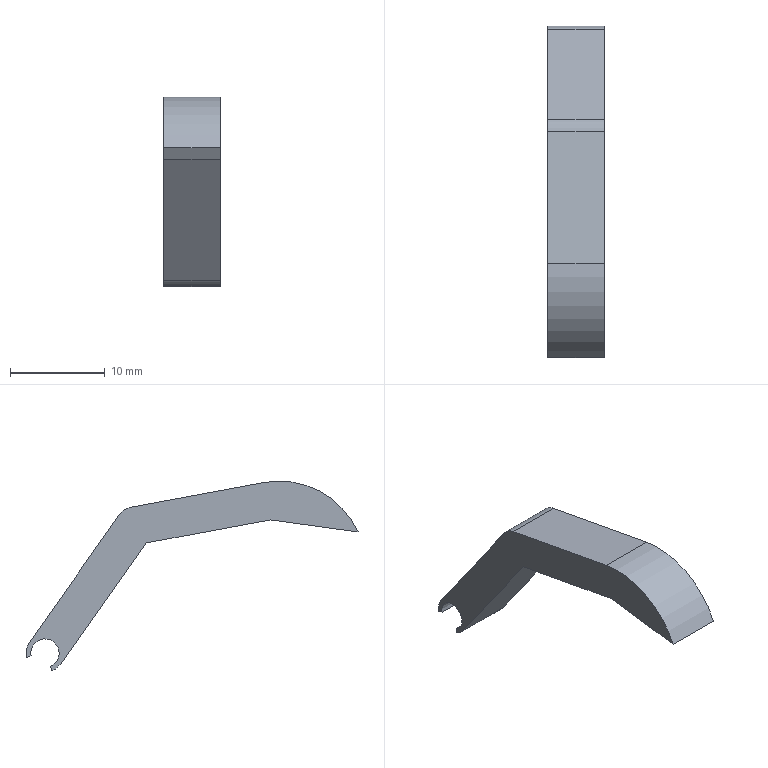Component | SolidWorks | Part14-10 | 1 solid | 17 faces | box 6 x 34.98 x 20 mm | volume 915 mm3 | plane 9 | cylinder 8 | commonest cylinder face diameters 4 x4 3 x3 18.228 x1
STEP:
#1=COLOUR_RGB('',0.7922,0.8196,0.9333);
#2=FILL_AREA_STYLE_COLOUR('',#1);
#3=FILL_AREA_STYLE('',(#2));
#4=SURFACE_STYLE_FILL_AREA(#3);
#5=SURFACE_SIDE_STYLE('',(#4));
#6=SURFACE_STYLE_USAGE(.BOTH.,#5);
#7=PRESENTATION_STYLE_ASSIGNMENT((#6));
#8=CARTESIAN_POINT('',(2.446,-0.3306,0.5502));
#9=VERTEX_POINT('',#8);
#10=CARTESIAN_POINT('',(2.446,-0.3522,0.5709));
#11=VERTEX_POINT('',#10);
#12=CARTESIAN_POINT('',(2.446,-0.2879,0.6163));
#13=DIRECTION('',(-1.,0.,0.));
#14=DIRECTION('',(0.,0.5427,0.84));
#15=AXIS2_PLACEMENT_3D('',#12,#13,#14);
#16=CIRCLE('',#15,0.07874);
#17=EDGE_CURVE('',#9,#11,#16,.T.);
#18=ORIENTED_EDGE('',*,*,#17,.F.);
#19=CARTESIAN_POINT('',(2.682,-0.3306,0.5502));
#20=VERTEX_POINT('',#19);
#21=CARTESIAN_POINT('',(2.446,-0.3306,0.5502));
#22=DIRECTION('',(1.,-0.,-0.));
#23=VECTOR('',#22,39.37);
#24=LINE('',#21,#23);
#25=EDGE_CURVE('',#9,#20,#24,.T.);
#26=ORIENTED_EDGE('',*,*,#25,.T.);
#27=CARTESIAN_POINT('',(2.682,-0.3522,0.5709));
#28=VERTEX_POINT('',#27);
#29=CARTESIAN_POINT('',(2.682,-0.2879,0.6163));
#30=DIRECTION('',(-1.,0.,0.));
#31=DIRECTION('',(0.,0.5427,0.84));
#32=AXIS2_PLACEMENT_3D('',#29,#30,#31);
#33=CIRCLE('',#32,0.07874);
#34=EDGE_CURVE('',#20,#28,#33,.T.);
#35=ORIENTED_EDGE('',*,*,#34,.T.);
#36=CARTESIAN_POINT('',(2.446,-0.3522,0.5709));
#37=DIRECTION('',(1.,-0.,-0.));
#38=VECTOR('',#37,39.37);
#39=LINE('',#36,#38);
#40=EDGE_CURVE('',#11,#28,#39,.T.);
#41=ORIENTED_EDGE('',*,*,#40,.F.);
#42=EDGE_LOOP('',(#18,#26,#35,#41));
#43=FACE_OUTER_BOUND('',#42,.T.);
#44=CARTESIAN_POINT('',(2.446,-0.2879,0.6163));
#45=DIRECTION('',(1.,-0.,-0.));
#46=DIRECTION('',(0.,-0.5427,-0.84));
#47=AXIS2_PLACEMENT_3D('',#44,#45,#46);
#48=CYLINDRICAL_SURFACE('',#47,0.07874);
#49=ADVANCED_FACE('',(#43),#48,.T.);
#50=CARTESIAN_POINT('',(2.446,-0.3199,0.5667));
#51=VERTEX_POINT('',#50);
#52=CARTESIAN_POINT('',(2.446,-0.2558,0.6659));
#53=VERTEX_POINT('',#52);
#54=CARTESIAN_POINT('',(2.446,-0.2879,0.6163));
#55=DIRECTION('',(-1.,0.,0.));
#56=DIRECTION('',(0.,0.5427,0.84));
#57=AXIS2_PLACEMENT_3D('',#54,#55,#56);
#58=CIRCLE('',#57,0.05906);
#59=EDGE_CURVE('',#51,#53,#58,.T.);
#60=ORIENTED_EDGE('',*,*,#59,.T.);
#61=CARTESIAN_POINT('',(2.682,-0.2558,0.6659));
#62=VERTEX_POINT('',#61);
#63=CARTESIAN_POINT('',(2.446,-0.2558,0.6659));
#64=DIRECTION('',(1.,-0.,-0.));
#65=VECTOR('',#64,39.37);
#66=LINE('',#63,#65);
#67=EDGE_CURVE('',#53,#62,#66,.T.);
#68=ORIENTED_EDGE('',*,*,#67,.T.);
#69=CARTESIAN_POINT('',(2.682,-0.3199,0.5667));
#70=VERTEX_POINT('',#69);
#71=CARTESIAN_POINT('',(2.682,-0.2879,0.6163));
#72=DIRECTION('',(-1.,0.,0.));
#73=DIRECTION('',(0.,0.5427,0.84));
#74=AXIS2_PLACEMENT_3D('',#71,#72,#73);
#75=CIRCLE('',#74,0.05906);
#76=EDGE_CURVE('',#70,#62,#75,.T.);
#77=ORIENTED_EDGE('',*,*,#76,.F.);
#78=CARTESIAN_POINT('',(2.446,-0.3199,0.5667));
#79=DIRECTION('',(1.,-0.,-0.));
#80=VECTOR('',#79,39.37);
#81=LINE('',#78,#80);
#82=EDGE_CURVE('',#51,#70,#81,.T.);
#83=ORIENTED_EDGE('',*,*,#82,.F.);
#84=EDGE_LOOP('',(#60,#68,#77,#83));
#85=FACE_OUTER_BOUND('',#84,.T.);
#86=CARTESIAN_POINT('',(2.446,-0.2879,0.6163));
#87=DIRECTION('',(1.,-0.,-0.));
#88=DIRECTION('',(0.,-0.5427,-0.84));
#89=AXIS2_PLACEMENT_3D('',#86,#87,#88);
#90=CYLINDRICAL_SURFACE('',#89,0.05906);
#91=ADVANCED_FACE('',(#85),#90,.F.);
#92=CARTESIAN_POINT('',(2.446,-0.3119,0.5624));
#93=VERTEX_POINT('',#92);
#94=CARTESIAN_POINT('',(2.446,-0.2879,0.6163));
#95=DIRECTION('',(-1.,0.,0.));
#96=DIRECTION('',(0.,0.5427,0.84));
#97=AXIS2_PLACEMENT_3D('',#94,#95,#96);
#98=CIRCLE('',#97,0.05906);
#99=EDGE_CURVE('',#93,#51,#98,.T.);
#100=ORIENTED_EDGE('',*,*,#99,.T.);
#101=ORIENTED_EDGE('',*,*,#82,.T.);
#102=CARTESIAN_POINT('',(2.682,-0.3119,0.5624));
#103=VERTEX_POINT('',#102);
#104=CARTESIAN_POINT('',(2.682,-0.2879,0.6163));
#105=DIRECTION('',(-1.,0.,0.));
#106=DIRECTION('',(0.,0.5427,0.84));
#107=AXIS2_PLACEMENT_3D('',#104,#105,#106);
#108=CIRCLE('',#107,0.05906);
#109=EDGE_CURVE('',#103,#70,#108,.T.);
#110=ORIENTED_EDGE('',*,*,#109,.F.);
#111=CARTESIAN_POINT('',(2.446,-0.3119,0.5624));
#112=DIRECTION('',(1.,-0.,-0.));
#113=VECTOR('',#112,39.37);
#114=LINE('',#111,#113);
#115=EDGE_CURVE('',#93,#103,#114,.T.);
#116=ORIENTED_EDGE('',*,*,#115,.F.);
#117=EDGE_LOOP('',(#100,#101,#110,#116));
#118=FACE_OUTER_BOUND('',#117,.T.);
#119=CARTESIAN_POINT('',(2.446,-0.2879,0.6163));
#120=DIRECTION('',(1.,-0.,-0.));
#121=DIRECTION('',(0.,-0.5427,-0.84));
#122=AXIS2_PLACEMENT_3D('',#119,#120,#121);
#123=CYLINDRICAL_SURFACE('',#122,0.05906);
#124=ADVANCED_FACE('',(#118),#123,.F.);
#125=CARTESIAN_POINT('',(2.682,-0.6463,1.222));
#126=VERTEX_POINT('',#125);
#127=CARTESIAN_POINT('',(2.682,-1.194,1.324));
#128=VERTEX_POINT('',#127);
#129=CARTESIAN_POINT('',(2.682,0.1495,1.074));
#130=DIRECTION('',(-0.,-0.9831,0.183));
#131=VECTOR('',#130,39.37);
#132=LINE('',#129,#131);
#133=EDGE_CURVE('',#126,#128,#132,.T.);
#134=ORIENTED_EDGE('',*,*,#133,.F.);
#135=CARTESIAN_POINT('',(2.446,-0.6463,1.222));
#136=VERTEX_POINT('',#135);
#137=CARTESIAN_POINT('',(2.446,-0.6463,1.222));
#138=DIRECTION('',(1.,-0.,-0.));
#139=VECTOR('',#138,39.37);
#140=LINE('',#137,#139);
#141=EDGE_CURVE('',#136,#126,#140,.T.);
#142=ORIENTED_EDGE('',*,*,#141,.F.);
#143=CARTESIAN_POINT('',(2.446,-1.194,1.324));
#144=VERTEX_POINT('',#143);
#145=CARTESIAN_POINT('',(2.446,0.1495,1.074));
#146=DIRECTION('',(-0.,-0.9831,0.183));
#147=VECTOR('',#146,39.37);
#148=LINE('',#145,#147);
#149=EDGE_CURVE('',#136,#144,#148,.T.);
#150=ORIENTED_EDGE('',*,*,#149,.T.);
#151=CARTESIAN_POINT('',(2.446,-1.194,1.324));
#152=DIRECTION('',(1.,-0.,-0.));
#153=VECTOR('',#152,39.37);
#154=LINE('',#151,#153);
#155=EDGE_CURVE('',#144,#128,#154,.T.);
#156=ORIENTED_EDGE('',*,*,#155,.T.);
#157=EDGE_LOOP('',(#134,#142,#150,#156));
#158=FACE_OUTER_BOUND('',#157,.T.);
#159=CARTESIAN_POINT('',(2.446,0.1495,1.074));
#160=DIRECTION('',(0.,0.183,0.9831));
#161=DIRECTION('',(0.,0.9831,-0.183));
#162=AXIS2_PLACEMENT_3D('',#159,#160,#161);
#163=PLANE('',#162);
#164=ADVANCED_FACE('',(#158),#163,.T.);
#165=CARTESIAN_POINT('',(2.682,-0.5963,1.19));
#166=VERTEX_POINT('',#165);
#167=CARTESIAN_POINT('',(2.682,-0.6607,1.145));
#168=DIRECTION('',(-1.,0.,0.));
#169=DIRECTION('',(0.,0.5427,0.84));
#170=AXIS2_PLACEMENT_3D('',#167,#168,#169);
#171=CIRCLE('',#170,0.07874);
#172=EDGE_CURVE('',#126,#166,#171,.T.);
#173=ORIENTED_EDGE('',*,*,#172,.T.);
#174=CARTESIAN_POINT('',(2.446,-0.5963,1.19));
#175=VERTEX_POINT('',#174);
#176=CARTESIAN_POINT('',(2.446,-0.5963,1.19));
#177=DIRECTION('',(1.,-0.,-0.));
#178=VECTOR('',#177,39.37);
#179=LINE('',#176,#178);
#180=EDGE_CURVE('',#175,#166,#179,.T.);
#181=ORIENTED_EDGE('',*,*,#180,.F.);
#182=CARTESIAN_POINT('',(2.446,-0.6607,1.145));
#183=DIRECTION('',(-1.,0.,0.));
#184=DIRECTION('',(0.,0.5427,0.84));
#185=AXIS2_PLACEMENT_3D('',#182,#183,#184);
#186=CIRCLE('',#185,0.07874);
#187=EDGE_CURVE('',#136,#175,#186,.T.);
#188=ORIENTED_EDGE('',*,*,#187,.F.);
#189=ORIENTED_EDGE('',*,*,#141,.T.);
#190=EDGE_LOOP('',(#173,#181,#188,#189));
#191=FACE_OUTER_BOUND('',#190,.T.);
#192=CARTESIAN_POINT('',(2.446,-0.6607,1.145));
#193=DIRECTION('',(1.,-0.,-0.));
#194=DIRECTION('',(0.,-0.5427,-0.84));
#195=AXIS2_PLACEMENT_3D('',#192,#193,#194);
#196=CYLINDRICAL_SURFACE('',#195,0.07874);
#197=ADVANCED_FACE('',(#191),#196,.T.);
#198=CARTESIAN_POINT('',(2.682,-0.2235,0.6617));
#199=VERTEX_POINT('',#198);
#200=CARTESIAN_POINT('',(2.682,0.241,0.003505));
#201=DIRECTION('',(0.,-0.5766,0.817));
#202=VECTOR('',#201,39.37);
#203=LINE('',#200,#202);
#204=EDGE_CURVE('',#199,#166,#203,.T.);
#205=ORIENTED_EDGE('',*,*,#204,.F.);
#206=CARTESIAN_POINT('',(2.446,-0.2235,0.6617));
#207=VERTEX_POINT('',#206);
#208=CARTESIAN_POINT('',(2.446,-0.2235,0.6617));
#209=DIRECTION('',(1.,-0.,-0.));
#210=VECTOR('',#209,39.37);
#211=LINE('',#208,#210);
#212=EDGE_CURVE('',#207,#199,#211,.T.);
#213=ORIENTED_EDGE('',*,*,#212,.F.);
#214=CARTESIAN_POINT('',(2.446,0.241,0.003505));
#215=DIRECTION('',(0.,-0.5766,0.817));
#216=VECTOR('',#215,39.37);
#217=LINE('',#214,#216);
#218=EDGE_CURVE('',#207,#175,#217,.T.);
#219=ORIENTED_EDGE('',*,*,#218,.T.);
#220=ORIENTED_EDGE('',*,*,#180,.T.);
#221=EDGE_LOOP('',(#205,#213,#219,#220));
#222=FACE_OUTER_BOUND('',#221,.T.);
#223=CARTESIAN_POINT('',(2.446,0.241,0.003505));
#224=DIRECTION('',(0.,0.817,0.5766));
#225=DIRECTION('',(-0.,0.5766,-0.817));
#226=AXIS2_PLACEMENT_3D('',#223,#224,#225);
#227=PLANE('',#226);
#228=ADVANCED_FACE('',(#222),#227,.T.);
#229=CARTESIAN_POINT('',(2.682,-0.2114,0.5977));
#230=VERTEX_POINT('',#229);
#231=CARTESIAN_POINT('',(2.682,-0.2879,0.6163));
#232=DIRECTION('',(-1.,0.,0.));
#233=DIRECTION('',(0.,0.5427,0.84));
#234=AXIS2_PLACEMENT_3D('',#231,#232,#233);
#235=CIRCLE('',#234,0.07874);
#236=EDGE_CURVE('',#199,#230,#235,.T.);
#237=ORIENTED_EDGE('',*,*,#236,.T.);
#238=CARTESIAN_POINT('',(2.446,-0.2114,0.5977));
#239=VERTEX_POINT('',#238);
#240=CARTESIAN_POINT('',(2.446,-0.2114,0.5977));
#241=DIRECTION('',(1.,-0.,-0.));
#242=VECTOR('',#241,39.37);
#243=LINE('',#240,#242);
#244=EDGE_CURVE('',#239,#230,#243,.T.);
#245=ORIENTED_EDGE('',*,*,#244,.F.);
#246=CARTESIAN_POINT('',(2.446,-0.2879,0.6163));
#247=DIRECTION('',(-1.,0.,0.));
#248=DIRECTION('',(0.,0.5427,0.84));
#249=AXIS2_PLACEMENT_3D('',#246,#247,#248);
#250=CIRCLE('',#249,0.07874);
#251=EDGE_CURVE('',#207,#239,#250,.T.);
#252=ORIENTED_EDGE('',*,*,#251,.F.);
#253=ORIENTED_EDGE('',*,*,#212,.T.);
#254=EDGE_LOOP('',(#237,#245,#252,#253));
#255=FACE_OUTER_BOUND('',#254,.T.);
#256=CARTESIAN_POINT('',(2.446,-0.2879,0.6163));
#257=DIRECTION('',(1.,-0.,-0.));
#258=DIRECTION('',(0.,-0.5427,-0.84));
#259=AXIS2_PLACEMENT_3D('',#256,#257,#258);
#260=CYLINDRICAL_SURFACE('',#259,0.07874);
#261=ADVANCED_FACE('',(#255),#260,.T.);
#262=CARTESIAN_POINT('',(2.682,-0.23,0.6047));
#263=VERTEX_POINT('',#262);
#264=CARTESIAN_POINT('',(2.682,0.1655,0.4558));
#265=DIRECTION('',(0.,0.9359,-0.3522));
#266=VECTOR('',#265,39.37);
#267=LINE('',#264,#266);
#268=EDGE_CURVE('',#263,#230,#267,.T.);
#269=ORIENTED_EDGE('',*,*,#268,.F.);
#270=CARTESIAN_POINT('',(2.446,-0.23,0.6047));
#271=VERTEX_POINT('',#270);
#272=CARTESIAN_POINT('',(2.446,-0.23,0.6047));
#273=DIRECTION('',(1.,-0.,-0.));
#274=VECTOR('',#273,39.37);
#275=LINE('',#272,#274);
#276=EDGE_CURVE('',#271,#263,#275,.T.);
#277=ORIENTED_EDGE('',*,*,#276,.F.);
#278=CARTESIAN_POINT('',(2.446,0.1655,0.4558));
#279=DIRECTION('',(0.,0.9359,-0.3522));
#280=VECTOR('',#279,39.37);
#281=LINE('',#278,#280);
#282=EDGE_CURVE('',#271,#239,#281,.T.);
#283=ORIENTED_EDGE('',*,*,#282,.T.);
#284=ORIENTED_EDGE('',*,*,#244,.T.);
#285=EDGE_LOOP('',(#269,#277,#283,#284));
#286=FACE_OUTER_BOUND('',#285,.T.);
#287=CARTESIAN_POINT('',(2.446,0.1655,0.4558));
#288=DIRECTION('',(-0.,-0.3522,-0.9359));
#289=DIRECTION('',(-0.,-0.9359,0.3522));
#290=AXIS2_PLACEMENT_3D('',#287,#288,#289);
#291=PLANE('',#290);
#292=ADVANCED_FACE('',(#286),#291,.T.);
#293=ORIENTED_EDGE('',*,*,#67,.F.);
#294=CARTESIAN_POINT('',(2.446,-0.2879,0.6163));
#295=DIRECTION('',(-1.,0.,0.));
#296=DIRECTION('',(0.,0.5427,0.84));
#297=AXIS2_PLACEMENT_3D('',#294,#295,#296);
#298=CIRCLE('',#297,0.05906);
#299=EDGE_CURVE('',#53,#271,#298,.T.);
#300=ORIENTED_EDGE('',*,*,#299,.T.);
#301=ORIENTED_EDGE('',*,*,#276,.T.);
#302=CARTESIAN_POINT('',(2.682,-0.2879,0.6163));
#303=DIRECTION('',(-1.,0.,0.));
#304=DIRECTION('',(0.,0.5427,0.84));
#305=AXIS2_PLACEMENT_3D('',#302,#303,#304);
#306=CIRCLE('',#305,0.05906);
#307=EDGE_CURVE('',#62,#263,#306,.T.);
#308=ORIENTED_EDGE('',*,*,#307,.F.);
#309=EDGE_LOOP('',(#293,#300,#301,#308));
#310=FACE_OUTER_BOUND('',#309,.T.);
#311=CARTESIAN_POINT('',(2.446,-0.2879,0.6163));
#312=DIRECTION('',(1.,-0.,-0.));
#313=DIRECTION('',(0.,-0.5427,-0.84));
#314=AXIS2_PLACEMENT_3D('',#311,#312,#313);
#315=CYLINDRICAL_SURFACE('',#314,0.05906);
#316=ADVANCED_FACE('',(#310),#315,.F.);
#317=CARTESIAN_POINT('',(2.682,-0.3156,0.5426));
#318=VERTEX_POINT('',#317);
#319=CARTESIAN_POINT('',(2.682,-0.4486,-0.1662));
#320=DIRECTION('',(-0.,-0.1844,-0.9829));
#321=VECTOR('',#320,39.37);
#322=LINE('',#319,#321);
#323=EDGE_CURVE('',#103,#318,#322,.T.);
#324=ORIENTED_EDGE('',*,*,#323,.T.);
#325=CARTESIAN_POINT('',(2.446,-0.3156,0.5426));
#326=VERTEX_POINT('',#325);
#327=CARTESIAN_POINT('',(2.446,-0.3156,0.5426));
#328=DIRECTION('',(1.,-0.,-0.));
#329=VECTOR('',#328,39.37);
#330=LINE('',#327,#329);
#331=EDGE_CURVE('',#326,#318,#330,.T.);
#332=ORIENTED_EDGE('',*,*,#331,.F.);
#333=CARTESIAN_POINT('',(2.446,-0.4486,-0.1662));
#334=DIRECTION('',(-0.,-0.1844,-0.9829));
#335=VECTOR('',#334,39.37);
#336=LINE('',#333,#335);
#337=EDGE_CURVE('',#93,#326,#336,.T.);
#338=ORIENTED_EDGE('',*,*,#337,.F.);
#339=ORIENTED_EDGE('',*,*,#115,.T.);
#340=EDGE_LOOP('',(#324,#332,#338,#339));
#341=FACE_OUTER_BOUND('',#340,.T.);
#342=CARTESIAN_POINT('',(2.446,-0.4486,-0.1662));
#343=DIRECTION('',(-0.,-0.9829,0.1844));
#344=DIRECTION('',(0.,0.1844,0.9829));
#345=AXIS2_PLACEMENT_3D('',#342,#343,#344);
#346=PLANE('',#345);
#347=ADVANCED_FACE('',(#341),#346,.F.);
#348=ORIENTED_EDGE('',*,*,#25,.F.);
#349=CARTESIAN_POINT('',(2.446,-0.2879,0.6163));
#350=DIRECTION('',(-1.,0.,0.));
#351=DIRECTION('',(0.,0.5427,0.84));
#352=AXIS2_PLACEMENT_3D('',#349,#350,#351);
#353=CIRCLE('',#352,0.07874);
#354=EDGE_CURVE('',#326,#9,#353,.T.);
#355=ORIENTED_EDGE('',*,*,#354,.F.);
#356=ORIENTED_EDGE('',*,*,#331,.T.);
#357=CARTESIAN_POINT('',(2.682,-0.2879,0.6163));
#358=DIRECTION('',(-1.,0.,0.));
#359=DIRECTION('',(0.,0.5427,0.84));
#360=AXIS2_PLACEMENT_3D('',#357,#358,#359);
#361=CIRCLE('',#360,0.07874);
#362=EDGE_CURVE('',#318,#20,#361,.T.);
#363=ORIENTED_EDGE('',*,*,#362,.T.);
#364=EDGE_LOOP('',(#348,#355,#356,#363));
#365=FACE_OUTER_BOUND('',#364,.T.);
#366=CARTESIAN_POINT('',(2.446,-0.2879,0.6163));
#367=DIRECTION('',(1.,-0.,-0.));
#368=DIRECTION('',(0.,-0.5427,-0.84));
#369=AXIS2_PLACEMENT_3D('',#366,#367,#368);
#370=CYLINDRICAL_SURFACE('',#369,0.07874);
#371=ADVANCED_FACE('',(#365),#370,.T.);
#372=CARTESIAN_POINT('',(2.682,-0.7066,1.073));
#373=VERTEX_POINT('',#372);
#374=CARTESIAN_POINT('',(2.682,0.1124,-0.0873));
#375=DIRECTION('',(0.,-0.5766,0.817));
#376=VECTOR('',#375,39.37);
#377=LINE('',#374,#376);
#378=EDGE_CURVE('',#28,#373,#377,.T.);
#379=ORIENTED_EDGE('',*,*,#378,.T.);
#380=CARTESIAN_POINT('',(2.446,-0.7066,1.073));
#381=VERTEX_POINT('',#380);
#382=CARTESIAN_POINT('',(2.446,-0.7066,1.073));
#383=DIRECTION('',(1.,-0.,-0.));
#384=VECTOR('',#383,39.37);
#385=LINE('',#382,#384);
#386=EDGE_CURVE('',#381,#373,#385,.T.);
#387=ORIENTED_EDGE('',*,*,#386,.F.);
#388=CARTESIAN_POINT('',(2.446,0.1124,-0.0873));
#389=DIRECTION('',(0.,-0.5766,0.817));
#390=VECTOR('',#389,39.37);
#391=LINE('',#388,#390);
#392=EDGE_CURVE('',#11,#381,#391,.T.);
#393=ORIENTED_EDGE('',*,*,#392,.F.);
#394=ORIENTED_EDGE('',*,*,#40,.T.);
#395=EDGE_LOOP('',(#379,#387,#393,#394));
#396=FACE_OUTER_BOUND('',#395,.T.);
#397=CARTESIAN_POINT('',(2.446,0.1124,-0.0873));
#398=DIRECTION('',(0.,0.817,0.5766));
#399=DIRECTION('',(-0.,0.5766,-0.817));
#400=AXIS2_PLACEMENT_3D('',#397,#398,#399);
#401=PLANE('',#400);
#402=ADVANCED_FACE('',(#396),#401,.F.);
#403=CARTESIAN_POINT('',(2.682,-1.223,1.169));
#404=VERTEX_POINT('',#403);
#405=CARTESIAN_POINT('',(2.682,0.1207,0.9191));
#406=DIRECTION('',(-0.,-0.9831,0.183));
#407=VECTOR('',#406,39.37);
#408=LINE('',#405,#407);
#409=EDGE_CURVE('',#373,#404,#408,.T.);
#410=ORIENTED_EDGE('',*,*,#409,.T.);
#411=CARTESIAN_POINT('',(2.446,-1.223,1.169));
#412=VERTEX_POINT('',#411);
#413=CARTESIAN_POINT('',(2.446,-1.223,1.169));
#414=DIRECTION('',(1.,-0.,-0.));
#415=VECTOR('',#414,39.37);
#416=LINE('',#413,#415);
#417=EDGE_CURVE('',#412,#404,#416,.T.);
#418=ORIENTED_EDGE('',*,*,#417,.F.);
#419=CARTESIAN_POINT('',(2.446,0.1207,0.9191));
#420=DIRECTION('',(-0.,-0.9831,0.183));
#421=VECTOR('',#420,39.37);
#422=LINE('',#419,#421);
#423=EDGE_CURVE('',#381,#412,#422,.T.);
#424=ORIENTED_EDGE('',*,*,#423,.F.);
#425=ORIENTED_EDGE('',*,*,#386,.T.);
#426=EDGE_LOOP('',(#410,#418,#424,#425));
#427=FACE_OUTER_BOUND('',#426,.T.);
#428=CARTESIAN_POINT('',(2.446,0.1207,0.9191));
#429=DIRECTION('',(0.,0.183,0.9831));
#430=DIRECTION('',(0.,0.9831,-0.183));
#431=AXIS2_PLACEMENT_3D('',#428,#429,#430);
#432=PLANE('',#431);
#433=ADVANCED_FACE('',(#427),#432,.F.);
#434=CARTESIAN_POINT('',(2.682,-1.586,1.119));
#435=VERTEX_POINT('',#434);
#436=CARTESIAN_POINT('',(2.682,-0.3035,1.295));
#437=DIRECTION('',(-0.,-0.9907,-0.136));
#438=VECTOR('',#437,39.37);
#439=LINE('',#436,#438);
#440=EDGE_CURVE('',#404,#435,#439,.T.);
#441=ORIENTED_EDGE('',*,*,#440,.T.);
#442=CARTESIAN_POINT('',(2.446,-1.586,1.119));
#443=VERTEX_POINT('',#442);
#444=CARTESIAN_POINT('',(2.446,-1.586,1.119));
#445=DIRECTION('',(1.,-0.,-0.));
#446=VECTOR('',#445,39.37);
#447=LINE('',#444,#446);
#448=EDGE_CURVE('',#443,#435,#447,.T.);
#449=ORIENTED_EDGE('',*,*,#448,.F.);
#450=CARTESIAN_POINT('',(2.446,-0.3035,1.295));
#451=DIRECTION('',(-0.,-0.9907,-0.136));
#452=VECTOR('',#451,39.37);
#453=LINE('',#450,#452);
#454=EDGE_CURVE('',#412,#443,#453,.T.);
#455=ORIENTED_EDGE('',*,*,#454,.F.);
#456=ORIENTED_EDGE('',*,*,#417,.T.);
#457=EDGE_LOOP('',(#441,#449,#455,#456));
#458=FACE_OUTER_BOUND('',#457,.T.);
#459=CARTESIAN_POINT('',(2.446,-0.3035,1.295));
#460=DIRECTION('',(0.,-0.136,0.9907));
#461=DIRECTION('',(0.,0.9907,0.136));
#462=AXIS2_PLACEMENT_3D('',#459,#460,#461);
#463=PLANE('',#462);
#464=ADVANCED_FACE('',(#458),#463,.F.);
#465=CARTESIAN_POINT('',(2.682,-1.26,0.9712));
#466=DIRECTION('',(-1.,0.,0.));
#467=DIRECTION('',(0.,0.5427,0.84));
#468=AXIS2_PLACEMENT_3D('',#465,#466,#467);
#469=CIRCLE('',#468,0.3588);
#470=EDGE_CURVE('',#435,#128,#469,.T.);
#471=ORIENTED_EDGE('',*,*,#470,.T.);
#472=ORIENTED_EDGE('',*,*,#155,.F.);
#473=CARTESIAN_POINT('',(2.446,-1.26,0.9712));
#474=DIRECTION('',(-1.,0.,0.));
#475=DIRECTION('',(0.,0.5427,0.84));
#476=AXIS2_PLACEMENT_3D('',#473,#474,#475);
#477=CIRCLE('',#476,0.3588);
#478=EDGE_CURVE('',#443,#144,#477,.T.);
#479=ORIENTED_EDGE('',*,*,#478,.F.);
#480=ORIENTED_EDGE('',*,*,#448,.T.);
#481=EDGE_LOOP('',(#471,#472,#479,#480));
#482=FACE_OUTER_BOUND('',#481,.T.);
#483=CARTESIAN_POINT('',(2.446,-1.26,0.9712));
#484=DIRECTION('',(1.,-0.,-0.));
#485=DIRECTION('',(0.,-0.5427,-0.84));
#486=AXIS2_PLACEMENT_3D('',#483,#484,#485);
#487=CYLINDRICAL_SURFACE('',#486,0.3588);
#488=ADVANCED_FACE('',(#482),#487,.T.);
#489=ORIENTED_EDGE('',*,*,#149,.F.);
#490=ORIENTED_EDGE('',*,*,#187,.T.);
#491=ORIENTED_EDGE('',*,*,#218,.F.);
#492=ORIENTED_EDGE('',*,*,#251,.T.);
#493=ORIENTED_EDGE('',*,*,#282,.F.);
#494=ORIENTED_EDGE('',*,*,#299,.F.);
#495=ORIENTED_EDGE('',*,*,#59,.F.);
#496=ORIENTED_EDGE('',*,*,#99,.F.);
#497=ORIENTED_EDGE('',*,*,#337,.T.);
#498=ORIENTED_EDGE('',*,*,#354,.T.);
#499=ORIENTED_EDGE('',*,*,#17,.T.);
#500=ORIENTED_EDGE('',*,*,#392,.T.);
#501=ORIENTED_EDGE('',*,*,#423,.T.);
#502=ORIENTED_EDGE('',*,*,#454,.T.);
#503=ORIENTED_EDGE('',*,*,#478,.T.);
#504=EDGE_LOOP('',(#489,#490,#491,#492,#493,#494,#495,#496,#497,#498,#499,#500,#501,#502,#503));
#505=FACE_OUTER_BOUND('',#504,.T.);
#506=CARTESIAN_POINT('',(2.446,-0.09369,-0.2327));
#507=DIRECTION('',(-1.,0.,0.));
#508=DIRECTION('',(0.,0.5427,0.84));
#509=AXIS2_PLACEMENT_3D('',#506,#507,#508);
#510=PLANE('',#509);
#511=ADVANCED_FACE('',(#505),#510,.T.);
#512=ORIENTED_EDGE('',*,*,#133,.T.);
#513=ORIENTED_EDGE('',*,*,#470,.F.);
#514=ORIENTED_EDGE('',*,*,#440,.F.);
#515=ORIENTED_EDGE('',*,*,#409,.F.);
#516=ORIENTED_EDGE('',*,*,#378,.F.);
#517=ORIENTED_EDGE('',*,*,#34,.F.);
#518=ORIENTED_EDGE('',*,*,#362,.F.);
#519=ORIENTED_EDGE('',*,*,#323,.F.);
#520=ORIENTED_EDGE('',*,*,#109,.T.);
#521=ORIENTED_EDGE('',*,*,#76,.T.);
#522=ORIENTED_EDGE('',*,*,#307,.T.);
#523=ORIENTED_EDGE('',*,*,#268,.T.);
#524=ORIENTED_EDGE('',*,*,#236,.F.);
#525=ORIENTED_EDGE('',*,*,#204,.T.);
#526=ORIENTED_EDGE('',*,*,#172,.F.);
#527=EDGE_LOOP('',(#512,#513,#514,#515,#516,#517,#518,#519,#520,#521,#522,#523,#524,#525,#526));
#528=FACE_OUTER_BOUND('',#527,.T.);
#529=CARTESIAN_POINT('',(2.682,-0.09369,-0.2327));
#530=DIRECTION('',(-1.,0.,0.));
#531=DIRECTION('',(0.,0.5427,0.84));
#532=AXIS2_PLACEMENT_3D('',#529,#530,#531);
#533=PLANE('',#532);
#534=ADVANCED_FACE('',(#528),#533,.F.);
#535=CLOSED_SHELL('',(#49,#91,#124,#164,#197,#228,#261,#292,#316,#347,#371,#402,#433,#464,#488,#511,#534));
#536=MANIFOLD_SOLID_BREP('',#535);
#537=STYLED_ITEM('',(#7),#536);
#538=(LENGTH_UNIT()NAMED_UNIT(*)SI_UNIT($,.METRE.));
#539=LENGTH_MEASURE_WITH_UNIT(LENGTH_MEASURE(0.0254),#538);
#540=DIMENSIONAL_EXPONENTS(1.,0.,0.,0.,0.,0.,0.);
#541=(CONVERSION_BASED_UNIT('',#539)LENGTH_UNIT()NAMED_UNIT(#540));
#542=UNCERTAINTY_MEASURE_WITH_UNIT(LENGTH_MEASURE(0.00001),#541,'','');
#543=(NAMED_UNIT(*)PLANE_ANGLE_UNIT()SI_UNIT($,.RADIAN.));
#544=(NAMED_UNIT(*)SI_UNIT($,.STERADIAN.)SOLID_ANGLE_UNIT());
#545=(GEOMETRIC_REPRESENTATION_CONTEXT(3)GLOBAL_UNCERTAINTY_ASSIGNED_CONTEXT((#542))GLOBAL_UNIT_ASSIGNED_CONTEXT((#541,#543,#544))REPRESENTATION_CONTEXT('',''));
#546=MECHANICAL_DESIGN_GEOMETRIC_PRESENTATION_REPRESENTATION('',(#537),#545);
#547=CARTESIAN_POINT('',(0.,0.,0.));
#548=DIRECTION('',(0.,0.,1.));
#549=DIRECTION('',(1.,0.,0.));
#550=AXIS2_PLACEMENT_3D('',#547,#548,#549);
#551=(LENGTH_UNIT()NAMED_UNIT(*)SI_UNIT($,.METRE.));
#552=LENGTH_MEASURE_WITH_UNIT(LENGTH_MEASURE(0.0254),#551);
#553=DIMENSIONAL_EXPONENTS(1.,0.,0.,0.,0.,0.,0.);
#554=(CONVERSION_BASED_UNIT('',#552)LENGTH_UNIT()NAMED_UNIT(#553));
#555=UNCERTAINTY_MEASURE_WITH_UNIT(LENGTH_MEASURE(0.00001),#554,'','');
#556=(NAMED_UNIT(*)PLANE_ANGLE_UNIT()SI_UNIT($,.RADIAN.));
#557=(NAMED_UNIT(*)SI_UNIT($,.STERADIAN.)SOLID_ANGLE_UNIT());
#558=(GEOMETRIC_REPRESENTATION_CONTEXT(3)GLOBAL_UNCERTAINTY_ASSIGNED_CONTEXT((#555))GLOBAL_UNIT_ASSIGNED_CONTEXT((#554,#556,#557))REPRESENTATION_CONTEXT('',''));
#559=ADVANCED_BREP_SHAPE_REPRESENTATION('',(#536,#550),#558);
#560=PRESENTATION_LAYER_ASSIGNMENT('','',(#537));